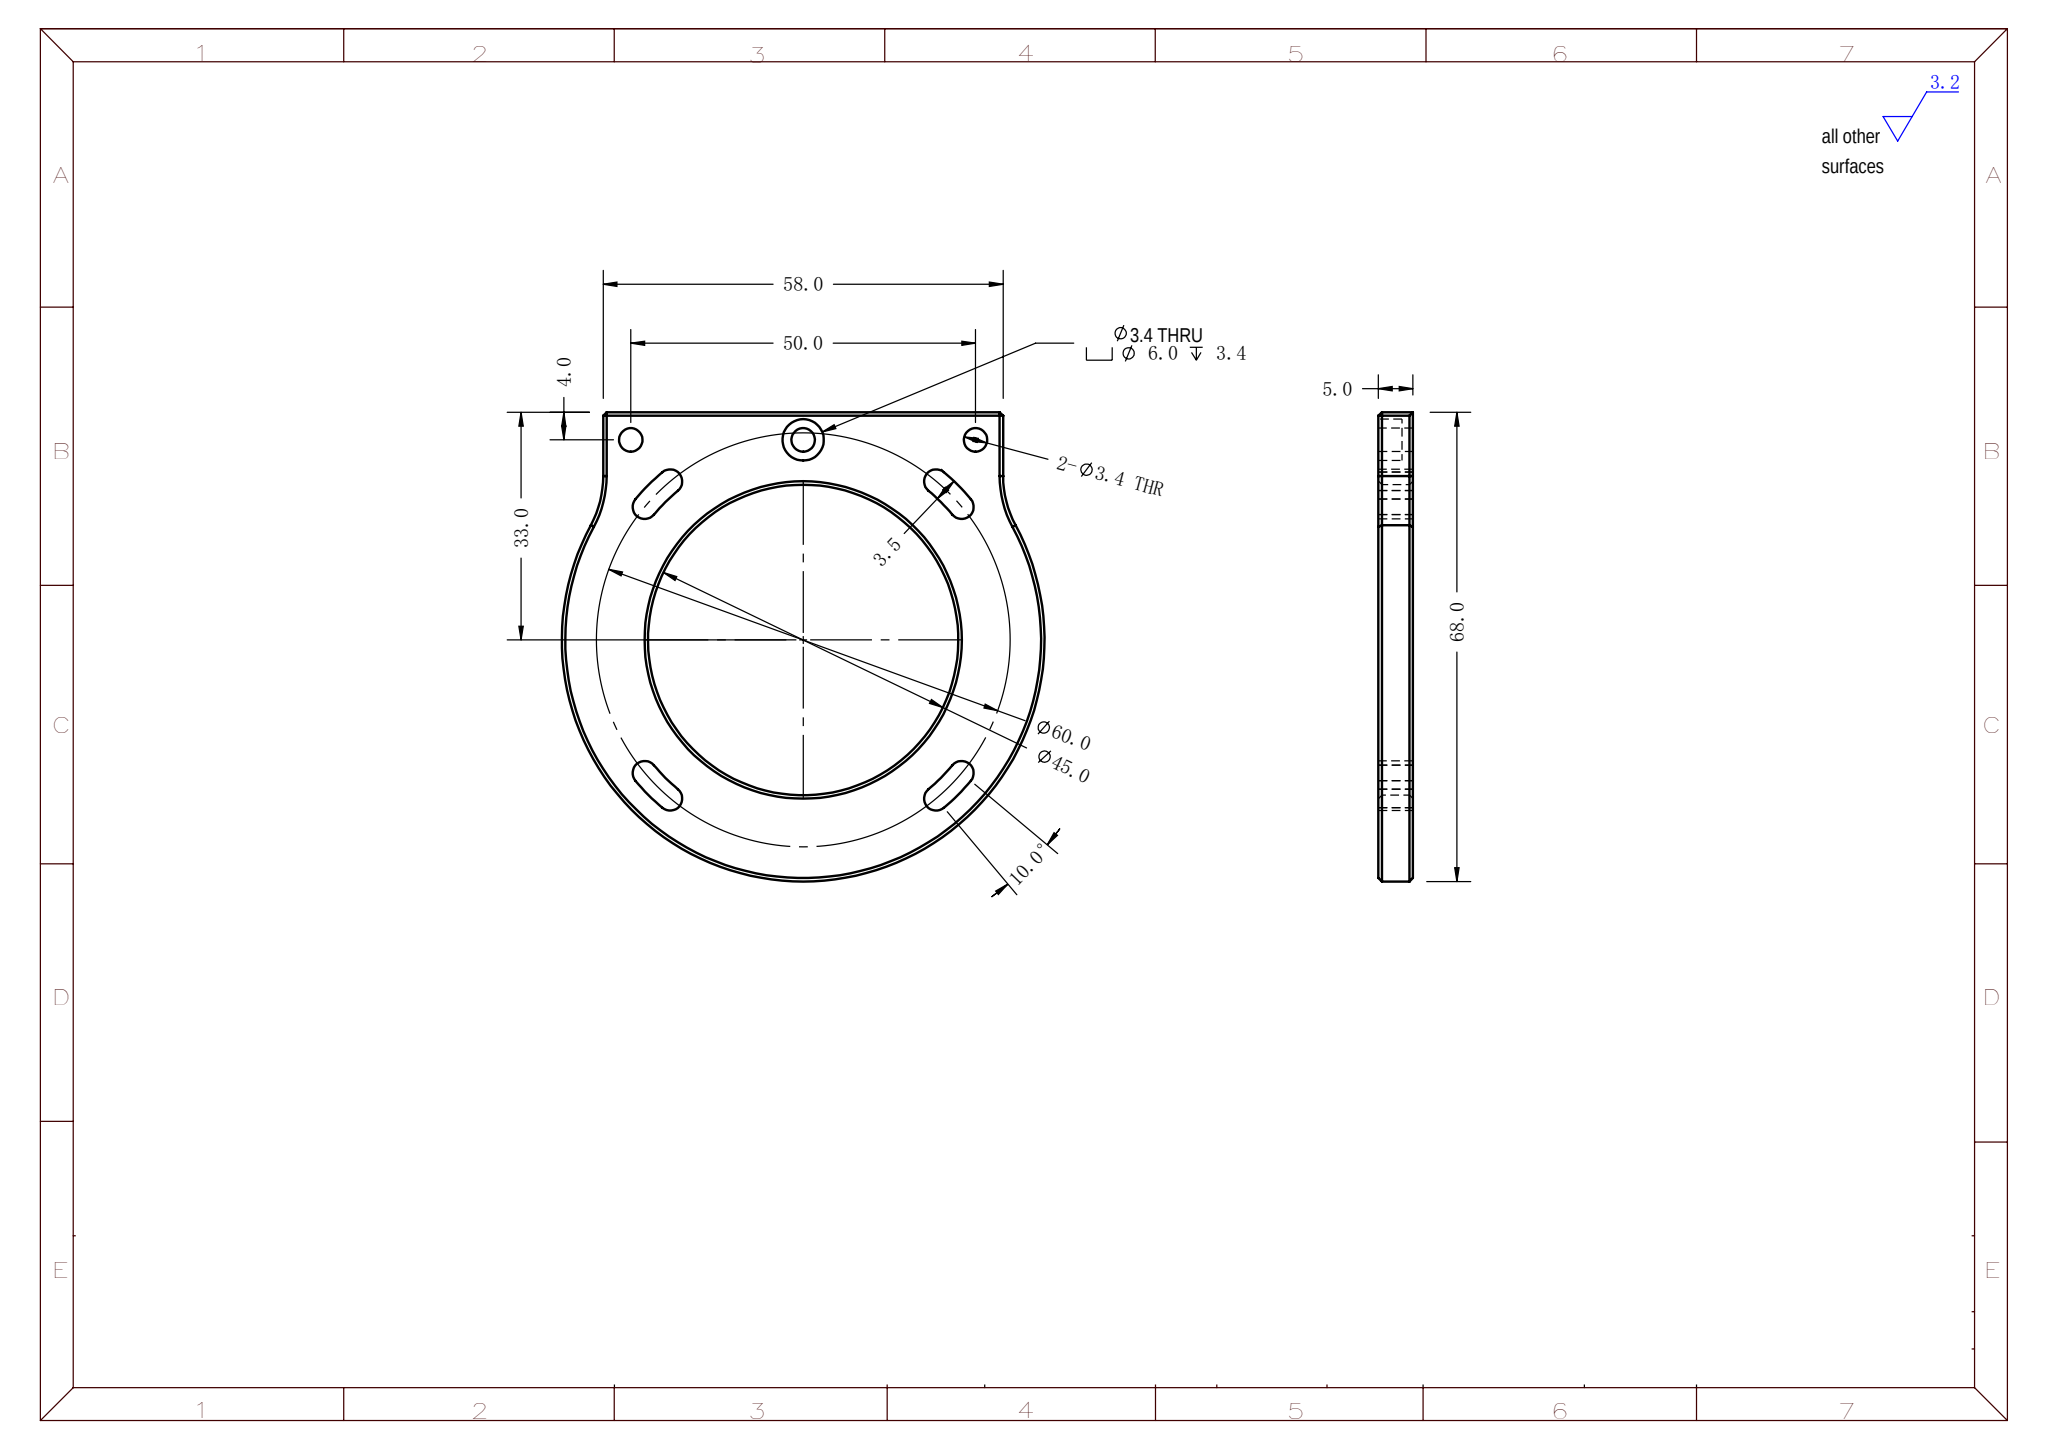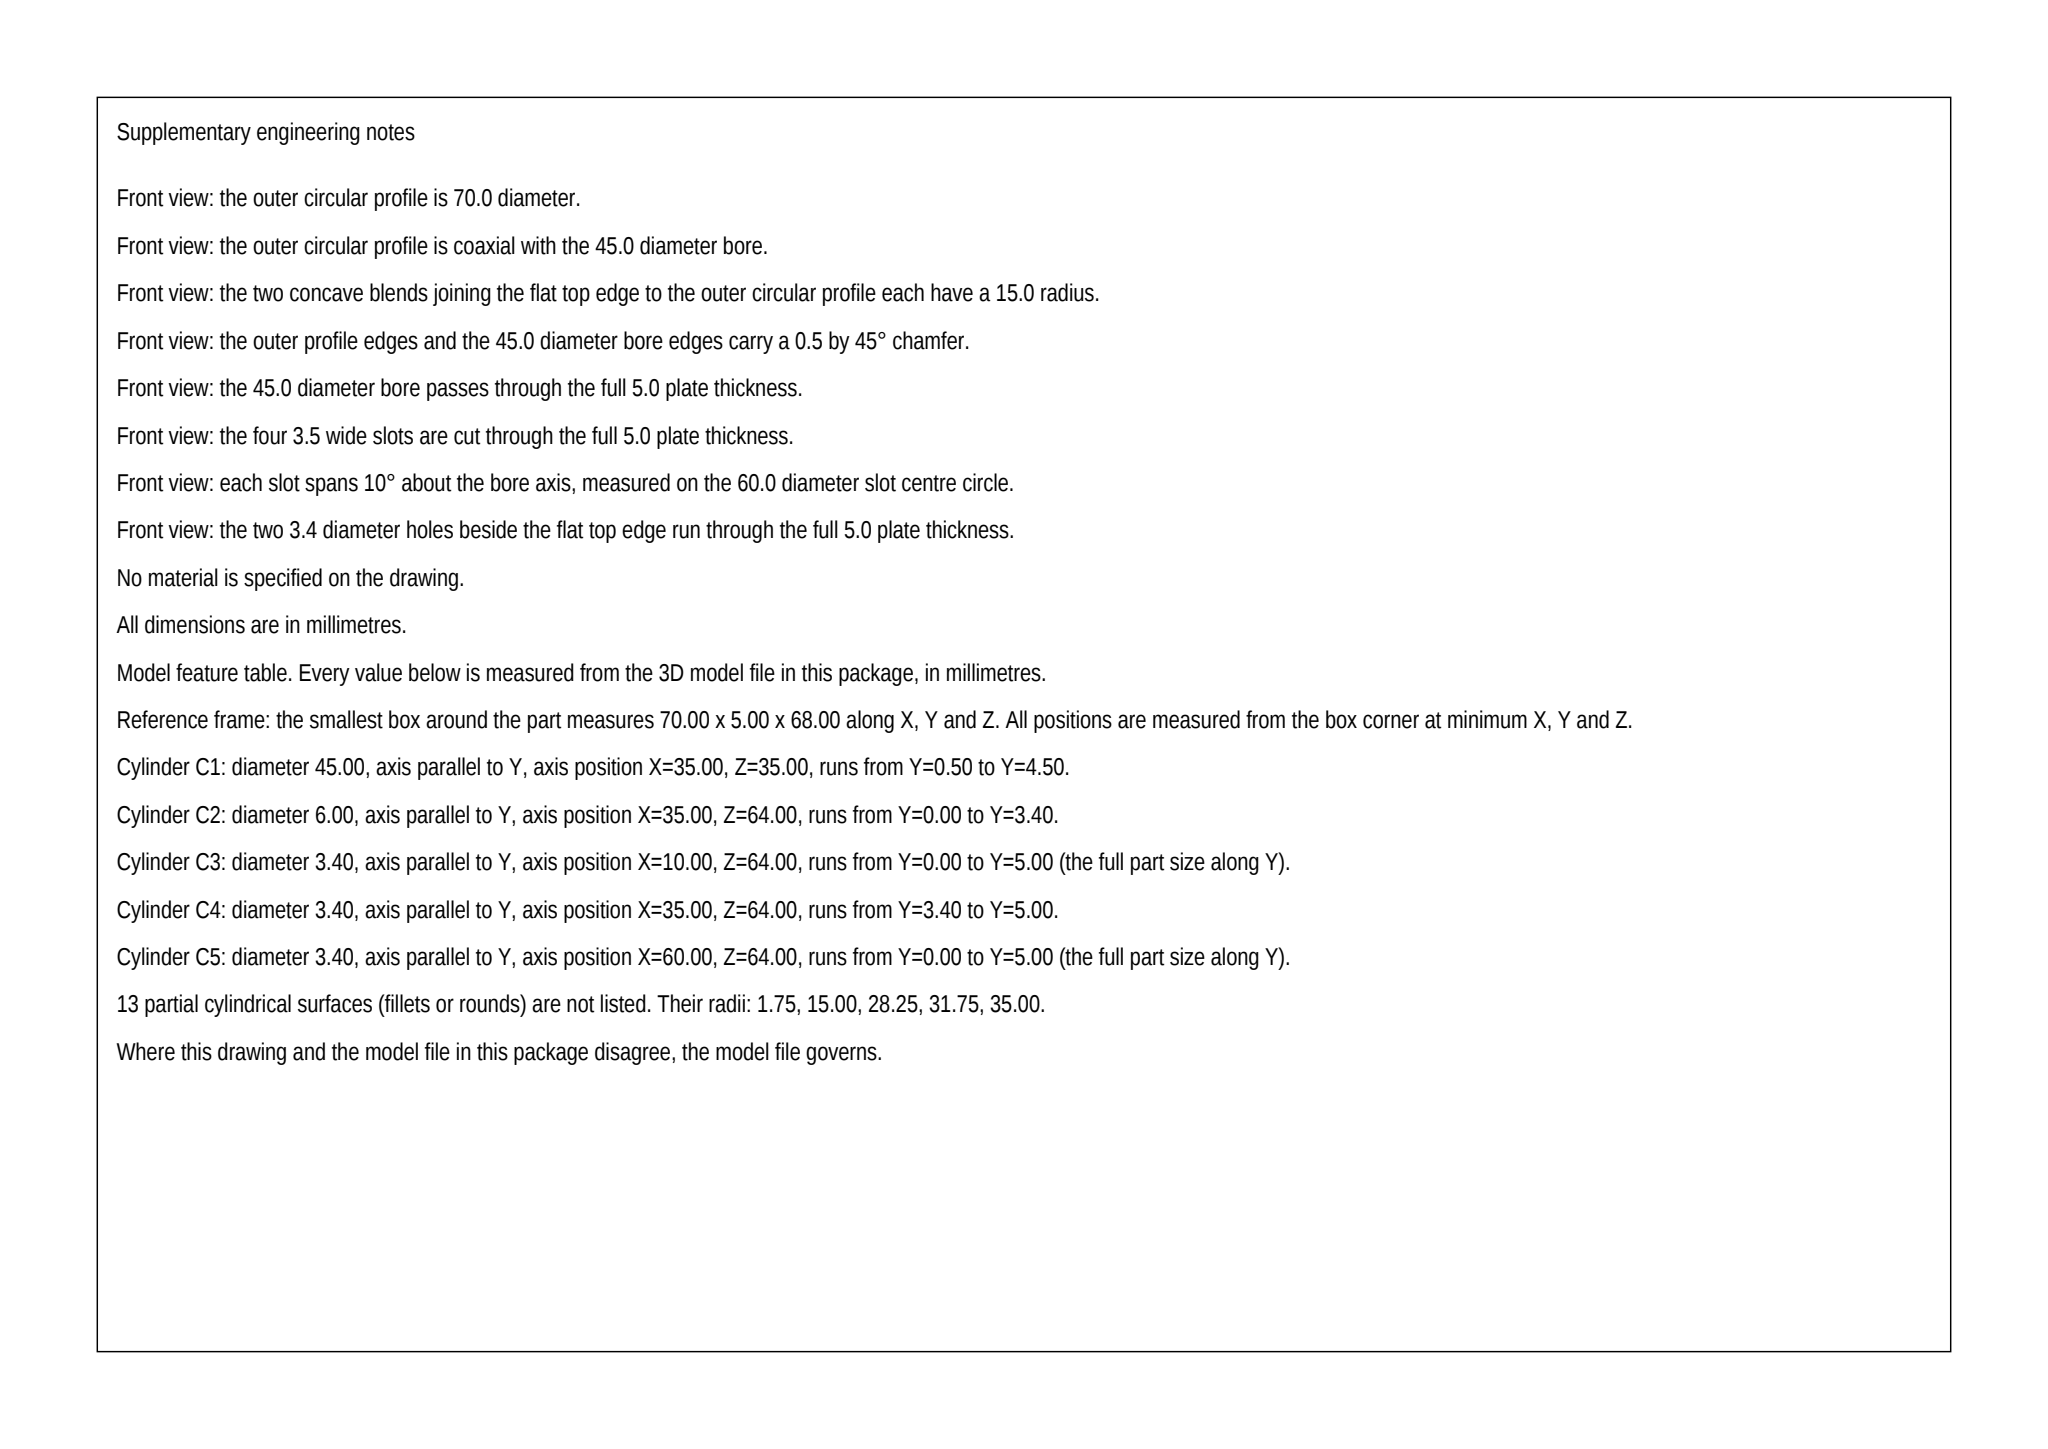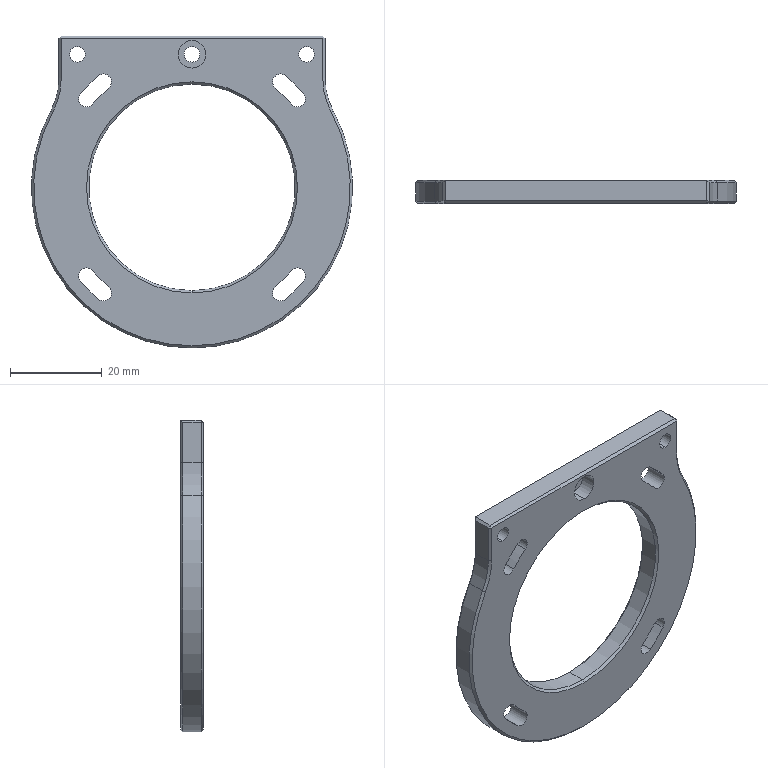Part | SolidWorks | mm | 1 solid | 60 faces | box 70 x 5 x 68 mm | volume 11203 mm3 | cylinder 34 | plane 15 | cone 11 | commonest cylinder face diameters 3.5 x12 3.4 x6 56.5 x4 63.5 x4 6 x2 45 x2 70 x2 30 x2
Drawing notes:
SIDE RELIEF R15: CTRS 44 EA SIDE VERT CL, 23.75 ABOVE HORIZ CL | from the solid: cyl dia30 axis y at x=-9 & 79, z=58.75; Ø70 ctr at (35,35)
4X ARC SLOT 3.5 WIDE x 10.0° ON Ø60 B.C., CTRS AT 45° EQ SP | from the solid: 3.5 dia end cyls at (12.02,15.72),(15.72,12.02) etc., r=30 from (35,35), ends ±5° about 45°
UNSPEC EDGES C0.5 x 45°: Ø45 BORE, Ø70 OD, R15 ARCS, BOTH FACES | from the solid: cones 90° incl, ref dia 45/46, 69/70, 30/31